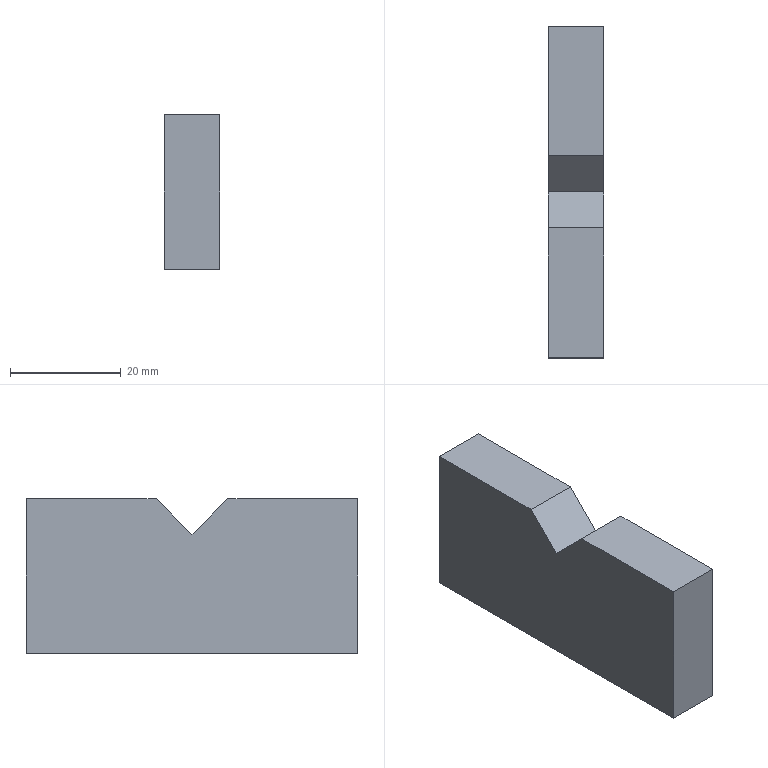Component | NX | REAR_BRACKET | 1 solid | 17 faces | box 10 x 60 x 28 mm | volume 15160 mm3 | plane 13 | cylinder 4 | commonest cylinder face diameters 5 x4
STEP:
#1=CARTESIAN_POINT('',(0.,0.,0.));
#2=DIRECTION('',(0.,0.,1.));
#3=DIRECTION('',(1.,0.,0.));
#4=AXIS2_PLACEMENT_3D('',#1,#2,#3);
#5=CARTESIAN_POINT('',(20.,-30.,34.5));
#6=VERTEX_POINT('',#5);
#7=CARTESIAN_POINT('',(20.,-6.5,34.5));
#8=VERTEX_POINT('',#7);
#9=CARTESIAN_POINT('',(20.,-30.,34.5));
#10=DIRECTION('',(0.,1.,-0.));
#11=VECTOR('',#10,1.);
#12=LINE('',#9,#11);
#13=CARTESIAN_POINT('',(30.,-30.,34.5));
#14=DIRECTION('',(0.,0.,1.));
#15=DIRECTION('',(0.,-1.,0.));
#16=AXIS2_PLACEMENT_3D('',#13,#14,#15);
#17=PLANE('',#16);
#18=CARTESIAN_POINT('',(0.,-10.));
#19=DIRECTION('',(-1.,0.));
#20=VECTOR('',#19,1.);
#21=LINE('',#18,#20);
#22=(GEOMETRIC_REPRESENTATION_CONTEXT(2)PARAMETRIC_REPRESENTATION_CONTEXT()REPRESENTATION_CONTEXT('',''));
#23=DEFINITIONAL_REPRESENTATION('',(#21),#22);
#24=PCURVE('',#17,#23);
#25=CARTESIAN_POINT('',(20.,0.,20.5));
#26=DIRECTION('',(-1.,0.,0.));
#27=DIRECTION('',(0.,0.,1.));
#28=AXIS2_PLACEMENT_3D('',#25,#26,#27);
#29=PLANE('',#28);
#30=CARTESIAN_POINT('',(14.,-30.));
#31=DIRECTION('',(-0.,1.));
#32=VECTOR('',#31,1.);
#33=LINE('',#30,#32);
#34=(GEOMETRIC_REPRESENTATION_CONTEXT(2)PARAMETRIC_REPRESENTATION_CONTEXT()REPRESENTATION_CONTEXT('',''));
#35=DEFINITIONAL_REPRESENTATION('',(#33),#34);
#36=PCURVE('',#29,#35);
#37=SURFACE_CURVE('',#12,(#24,#36),.PCURVE_S1.);
#38=EDGE_CURVE('',#6,#8,#37,.T.);
#39=ORIENTED_EDGE('',*,*,#38,.F.);
#40=CARTESIAN_POINT('',(30.,-30.,34.5));
#41=VERTEX_POINT('',#40);
#42=CARTESIAN_POINT('',(30.,-30.,34.5));
#43=DIRECTION('',(-1.,0.,0.));
#44=VECTOR('',#43,1.);
#45=LINE('',#42,#44);
#46=CARTESIAN_POINT('',(0.,0.));
#47=DIRECTION('',(0.,-1.));
#48=VECTOR('',#47,1.);
#49=LINE('',#46,#48);
#50=(GEOMETRIC_REPRESENTATION_CONTEXT(2)PARAMETRIC_REPRESENTATION_CONTEXT()REPRESENTATION_CONTEXT('',''));
#51=DEFINITIONAL_REPRESENTATION('',(#49),#50);
#52=PCURVE('',#17,#51);
#53=CARTESIAN_POINT('',(30.,-30.,6.5));
#54=DIRECTION('',(0.,-1.,0.));
#55=DIRECTION('',(0.,0.,-1.));
#56=AXIS2_PLACEMENT_3D('',#53,#54,#55);
#57=PLANE('',#56);
#58=CARTESIAN_POINT('',(-28.,0.));
#59=DIRECTION('',(0.,-1.));
#60=VECTOR('',#59,1.);
#61=LINE('',#58,#60);
#62=(GEOMETRIC_REPRESENTATION_CONTEXT(2)PARAMETRIC_REPRESENTATION_CONTEXT()REPRESENTATION_CONTEXT('',''));
#63=DEFINITIONAL_REPRESENTATION('',(#61),#62);
#64=PCURVE('',#57,#63);
#65=SURFACE_CURVE('',#45,(#52,#64),.PCURVE_S1.);
#66=EDGE_CURVE('',#41,#6,#65,.T.);
#67=ORIENTED_EDGE('',*,*,#66,.F.);
#68=CARTESIAN_POINT('',(30.,-6.5,34.5));
#69=VERTEX_POINT('',#68);
#70=CARTESIAN_POINT('',(30.,-30.,34.5));
#71=DIRECTION('',(0.,1.,-0.));
#72=VECTOR('',#71,1.);
#73=LINE('',#70,#72);
#74=CARTESIAN_POINT('',(0.,0.));
#75=DIRECTION('',(-1.,0.));
#76=VECTOR('',#75,1.);
#77=LINE('',#74,#76);
#78=(GEOMETRIC_REPRESENTATION_CONTEXT(2)PARAMETRIC_REPRESENTATION_CONTEXT()REPRESENTATION_CONTEXT('',''));
#79=DEFINITIONAL_REPRESENTATION('',(#77),#78);
#80=PCURVE('',#17,#79);
#81=CARTESIAN_POINT('',(30.,0.,20.5));
#82=DIRECTION('',(-1.,0.,0.));
#83=DIRECTION('',(0.,0.,1.));
#84=AXIS2_PLACEMENT_3D('',#81,#82,#83);
#85=PLANE('',#84);
#86=CARTESIAN_POINT('',(14.,-30.));
#87=DIRECTION('',(-0.,1.));
#88=VECTOR('',#87,1.);
#89=LINE('',#86,#88);
#90=(GEOMETRIC_REPRESENTATION_CONTEXT(2)PARAMETRIC_REPRESENTATION_CONTEXT()REPRESENTATION_CONTEXT('',''));
#91=DEFINITIONAL_REPRESENTATION('',(#89),#90);
#92=PCURVE('',#85,#91);
#93=SURFACE_CURVE('',#73,(#80,#92),.PCURVE_S1.);
#94=EDGE_CURVE('',#41,#69,#93,.T.);
#95=ORIENTED_EDGE('',*,*,#94,.T.);
#96=CARTESIAN_POINT('',(30.,-6.5,34.5));
#97=DIRECTION('',(-1.,0.,0.));
#98=VECTOR('',#97,1.);
#99=LINE('',#96,#98);
#100=CARTESIAN_POINT('',(-23.5,0.));
#101=DIRECTION('',(0.,-1.));
#102=VECTOR('',#101,1.);
#103=LINE('',#100,#102);
#104=(GEOMETRIC_REPRESENTATION_CONTEXT(2)PARAMETRIC_REPRESENTATION_CONTEXT()REPRESENTATION_CONTEXT('',''));
#105=DEFINITIONAL_REPRESENTATION('',(#103),#104);
#106=PCURVE('',#17,#105);
#107=CARTESIAN_POINT('',(30.,-6.5,34.5));
#108=DIRECTION('',(0.,0.7071,0.7071));
#109=DIRECTION('',(0.,-0.7071,0.7071));
#110=AXIS2_PLACEMENT_3D('',#107,#108,#109);
#111=PLANE('',#110);
#112=CARTESIAN_POINT('',(0.,0.));
#113=DIRECTION('',(0.,-1.));
#114=VECTOR('',#113,1.);
#115=LINE('',#112,#114);
#116=(GEOMETRIC_REPRESENTATION_CONTEXT(2)PARAMETRIC_REPRESENTATION_CONTEXT()REPRESENTATION_CONTEXT('',''));
#117=DEFINITIONAL_REPRESENTATION('',(#115),#116);
#118=PCURVE('',#111,#117);
#119=SURFACE_CURVE('',#99,(#106,#118),.PCURVE_S1.);
#120=EDGE_CURVE('',#69,#8,#119,.T.);
#121=ORIENTED_EDGE('',*,*,#120,.T.);
#122=EDGE_LOOP('',(#39,#67,#95,#121));
#123=FACE_BOUND('',#122,.T.);
#124=ADVANCED_FACE('',(#123),#17,.T.);
#125=CARTESIAN_POINT('',(20.,0.,28.));
#126=VERTEX_POINT('',#125);
#127=CARTESIAN_POINT('',(20.,-6.5,34.5));
#128=DIRECTION('',(0.,0.7071,-0.7071));
#129=VECTOR('',#128,1.);
#130=LINE('',#127,#129);
#131=CARTESIAN_POINT('',(0.,-10.));
#132=DIRECTION('',(-1.,0.));
#133=VECTOR('',#132,1.);
#134=LINE('',#131,#133);
#135=(GEOMETRIC_REPRESENTATION_CONTEXT(2)PARAMETRIC_REPRESENTATION_CONTEXT()REPRESENTATION_CONTEXT('',''));
#136=DEFINITIONAL_REPRESENTATION('',(#134),#135);
#137=PCURVE('',#111,#136);
#138=CARTESIAN_POINT('',(14.,-6.5));
#139=DIRECTION('',(-0.7071,0.7071));
#140=VECTOR('',#139,1.);
#141=LINE('',#138,#140);
#142=(GEOMETRIC_REPRESENTATION_CONTEXT(2)PARAMETRIC_REPRESENTATION_CONTEXT()REPRESENTATION_CONTEXT('',''));
#143=DEFINITIONAL_REPRESENTATION('',(#141),#142);
#144=PCURVE('',#29,#143);
#145=SURFACE_CURVE('',#130,(#137,#144),.PCURVE_S1.);
#146=EDGE_CURVE('',#8,#126,#145,.T.);
#147=ORIENTED_EDGE('',*,*,#146,.F.);
#148=ORIENTED_EDGE('',*,*,#120,.F.);
#149=CARTESIAN_POINT('',(30.,0.,28.));
#150=VERTEX_POINT('',#149);
#151=CARTESIAN_POINT('',(30.,-6.5,34.5));
#152=DIRECTION('',(0.,0.7071,-0.7071));
#153=VECTOR('',#152,1.);
#154=LINE('',#151,#153);
#155=CARTESIAN_POINT('',(0.,0.));
#156=DIRECTION('',(-1.,0.));
#157=VECTOR('',#156,1.);
#158=LINE('',#155,#157);
#159=(GEOMETRIC_REPRESENTATION_CONTEXT(2)PARAMETRIC_REPRESENTATION_CONTEXT()REPRESENTATION_CONTEXT('',''));
#160=DEFINITIONAL_REPRESENTATION('',(#158),#159);
#161=PCURVE('',#111,#160);
#162=CARTESIAN_POINT('',(14.,-6.5));
#163=DIRECTION('',(-0.7071,0.7071));
#164=VECTOR('',#163,1.);
#165=LINE('',#162,#164);
#166=(GEOMETRIC_REPRESENTATION_CONTEXT(2)PARAMETRIC_REPRESENTATION_CONTEXT()REPRESENTATION_CONTEXT('',''));
#167=DEFINITIONAL_REPRESENTATION('',(#165),#166);
#168=PCURVE('',#85,#167);
#169=SURFACE_CURVE('',#154,(#161,#168),.PCURVE_S1.);
#170=EDGE_CURVE('',#69,#150,#169,.T.);
#171=ORIENTED_EDGE('',*,*,#170,.T.);
#172=CARTESIAN_POINT('',(30.,0.,28.));
#173=DIRECTION('',(-1.,0.,0.));
#174=VECTOR('',#173,1.);
#175=LINE('',#172,#174);
#176=CARTESIAN_POINT('',(-9.192,0.));
#177=DIRECTION('',(0.,-1.));
#178=VECTOR('',#177,1.);
#179=LINE('',#176,#178);
#180=(GEOMETRIC_REPRESENTATION_CONTEXT(2)PARAMETRIC_REPRESENTATION_CONTEXT()REPRESENTATION_CONTEXT('',''));
#181=DEFINITIONAL_REPRESENTATION('',(#179),#180);
#182=PCURVE('',#111,#181);
#183=CARTESIAN_POINT('',(30.,0.,28.));
#184=DIRECTION('',(0.,-0.7071,0.7071));
#185=DIRECTION('',(0.,-0.7071,-0.7071));
#186=AXIS2_PLACEMENT_3D('',#183,#184,#185);
#187=PLANE('',#186);
#188=CARTESIAN_POINT('',(0.,0.));
#189=DIRECTION('',(0.,-1.));
#190=VECTOR('',#189,1.);
#191=LINE('',#188,#190);
#192=(GEOMETRIC_REPRESENTATION_CONTEXT(2)PARAMETRIC_REPRESENTATION_CONTEXT()REPRESENTATION_CONTEXT('',''));
#193=DEFINITIONAL_REPRESENTATION('',(#191),#192);
#194=PCURVE('',#187,#193);
#195=SURFACE_CURVE('',#175,(#182,#194),.PCURVE_S1.);
#196=EDGE_CURVE('',#150,#126,#195,.T.);
#197=ORIENTED_EDGE('',*,*,#196,.T.);
#198=EDGE_LOOP('',(#147,#148,#171,#197));
#199=FACE_BOUND('',#198,.T.);
#200=ADVANCED_FACE('',(#199),#111,.T.);
#201=CARTESIAN_POINT('',(20.,6.5,34.5));
#202=VERTEX_POINT('',#201);
#203=CARTESIAN_POINT('',(20.,0.,28.));
#204=DIRECTION('',(0.,0.7071,0.7071));
#205=VECTOR('',#204,1.);
#206=LINE('',#203,#205);
#207=CARTESIAN_POINT('',(0.,-10.));
#208=DIRECTION('',(-1.,0.));
#209=VECTOR('',#208,1.);
#210=LINE('',#207,#209);
#211=(GEOMETRIC_REPRESENTATION_CONTEXT(2)PARAMETRIC_REPRESENTATION_CONTEXT()REPRESENTATION_CONTEXT('',''));
#212=DEFINITIONAL_REPRESENTATION('',(#210),#211);
#213=PCURVE('',#187,#212);
#214=CARTESIAN_POINT('',(7.5,0.));
#215=DIRECTION('',(0.7071,0.7071));
#216=VECTOR('',#215,1.);
#217=LINE('',#214,#216);
#218=(GEOMETRIC_REPRESENTATION_CONTEXT(2)PARAMETRIC_REPRESENTATION_CONTEXT()REPRESENTATION_CONTEXT('',''));
#219=DEFINITIONAL_REPRESENTATION('',(#217),#218);
#220=PCURVE('',#29,#219);
#221=SURFACE_CURVE('',#206,(#213,#220),.PCURVE_S1.);
#222=EDGE_CURVE('',#126,#202,#221,.T.);
#223=ORIENTED_EDGE('',*,*,#222,.F.);
#224=ORIENTED_EDGE('',*,*,#196,.F.);
#225=CARTESIAN_POINT('',(30.,6.5,34.5));
#226=VERTEX_POINT('',#225);
#227=CARTESIAN_POINT('',(30.,0.,28.));
#228=DIRECTION('',(0.,0.7071,0.7071));
#229=VECTOR('',#228,1.);
#230=LINE('',#227,#229);
#231=CARTESIAN_POINT('',(0.,0.));
#232=DIRECTION('',(-1.,0.));
#233=VECTOR('',#232,1.);
#234=LINE('',#231,#233);
#235=(GEOMETRIC_REPRESENTATION_CONTEXT(2)PARAMETRIC_REPRESENTATION_CONTEXT()REPRESENTATION_CONTEXT('',''));
#236=DEFINITIONAL_REPRESENTATION('',(#234),#235);
#237=PCURVE('',#187,#236);
#238=CARTESIAN_POINT('',(7.5,0.));
#239=DIRECTION('',(0.7071,0.7071));
#240=VECTOR('',#239,1.);
#241=LINE('',#238,#240);
#242=(GEOMETRIC_REPRESENTATION_CONTEXT(2)PARAMETRIC_REPRESENTATION_CONTEXT()REPRESENTATION_CONTEXT('',''));
#243=DEFINITIONAL_REPRESENTATION('',(#241),#242);
#244=PCURVE('',#85,#243);
#245=SURFACE_CURVE('',#230,(#237,#244),.PCURVE_S1.);
#246=EDGE_CURVE('',#150,#226,#245,.T.);
#247=ORIENTED_EDGE('',*,*,#246,.T.);
#248=CARTESIAN_POINT('',(30.,6.5,34.5));
#249=DIRECTION('',(-1.,0.,0.));
#250=VECTOR('',#249,1.);
#251=LINE('',#248,#250);
#252=CARTESIAN_POINT('',(-9.192,0.));
#253=DIRECTION('',(0.,-1.));
#254=VECTOR('',#253,1.);
#255=LINE('',#252,#254);
#256=(GEOMETRIC_REPRESENTATION_CONTEXT(2)PARAMETRIC_REPRESENTATION_CONTEXT()REPRESENTATION_CONTEXT('',''));
#257=DEFINITIONAL_REPRESENTATION('',(#255),#256);
#258=PCURVE('',#187,#257);
#259=CARTESIAN_POINT('',(30.,6.5,34.5));
#260=DIRECTION('',(0.,-0.,1.));
#261=DIRECTION('',(0.,-1.,-0.));
#262=AXIS2_PLACEMENT_3D('',#259,#260,#261);
#263=PLANE('',#262);
#264=CARTESIAN_POINT('',(0.,0.));
#265=DIRECTION('',(0.,-1.));
#266=VECTOR('',#265,1.);
#267=LINE('',#264,#266);
#268=(GEOMETRIC_REPRESENTATION_CONTEXT(2)PARAMETRIC_REPRESENTATION_CONTEXT()REPRESENTATION_CONTEXT('',''));
#269=DEFINITIONAL_REPRESENTATION('',(#267),#268);
#270=PCURVE('',#263,#269);
#271=SURFACE_CURVE('',#251,(#258,#270),.PCURVE_S1.);
#272=EDGE_CURVE('',#226,#202,#271,.T.);
#273=ORIENTED_EDGE('',*,*,#272,.T.);
#274=EDGE_LOOP('',(#223,#224,#247,#273));
#275=FACE_BOUND('',#274,.T.);
#276=ADVANCED_FACE('',(#275),#187,.T.);
#277=CARTESIAN_POINT('',(20.,30.,34.5));
#278=VERTEX_POINT('',#277);
#279=CARTESIAN_POINT('',(20.,6.5,34.5));
#280=DIRECTION('',(0.,1.,0.));
#281=VECTOR('',#280,1.);
#282=LINE('',#279,#281);
#283=CARTESIAN_POINT('',(0.,-10.));
#284=DIRECTION('',(-1.,0.));
#285=VECTOR('',#284,1.);
#286=LINE('',#283,#285);
#287=(GEOMETRIC_REPRESENTATION_CONTEXT(2)PARAMETRIC_REPRESENTATION_CONTEXT()REPRESENTATION_CONTEXT('',''));
#288=DEFINITIONAL_REPRESENTATION('',(#286),#287);
#289=PCURVE('',#263,#288);
#290=CARTESIAN_POINT('',(14.,6.5));
#291=DIRECTION('',(0.,1.));
#292=VECTOR('',#291,1.);
#293=LINE('',#290,#292);
#294=(GEOMETRIC_REPRESENTATION_CONTEXT(2)PARAMETRIC_REPRESENTATION_CONTEXT()REPRESENTATION_CONTEXT('',''));
#295=DEFINITIONAL_REPRESENTATION('',(#293),#294);
#296=PCURVE('',#29,#295);
#297=SURFACE_CURVE('',#282,(#289,#296),.PCURVE_S1.);
#298=EDGE_CURVE('',#202,#278,#297,.T.);
#299=ORIENTED_EDGE('',*,*,#298,.F.);
#300=ORIENTED_EDGE('',*,*,#272,.F.);
#301=CARTESIAN_POINT('',(30.,30.,34.5));
#302=VERTEX_POINT('',#301);
#303=CARTESIAN_POINT('',(30.,6.5,34.5));
#304=DIRECTION('',(0.,1.,0.));
#305=VECTOR('',#304,1.);
#306=LINE('',#303,#305);
#307=CARTESIAN_POINT('',(0.,0.));
#308=DIRECTION('',(-1.,0.));
#309=VECTOR('',#308,1.);
#310=LINE('',#307,#309);
#311=(GEOMETRIC_REPRESENTATION_CONTEXT(2)PARAMETRIC_REPRESENTATION_CONTEXT()REPRESENTATION_CONTEXT('',''));
#312=DEFINITIONAL_REPRESENTATION('',(#310),#311);
#313=PCURVE('',#263,#312);
#314=CARTESIAN_POINT('',(14.,6.5));
#315=DIRECTION('',(0.,1.));
#316=VECTOR('',#315,1.);
#317=LINE('',#314,#316);
#318=(GEOMETRIC_REPRESENTATION_CONTEXT(2)PARAMETRIC_REPRESENTATION_CONTEXT()REPRESENTATION_CONTEXT('',''));
#319=DEFINITIONAL_REPRESENTATION('',(#317),#318);
#320=PCURVE('',#85,#319);
#321=SURFACE_CURVE('',#306,(#313,#320),.PCURVE_S1.);
#322=EDGE_CURVE('',#226,#302,#321,.T.);
#323=ORIENTED_EDGE('',*,*,#322,.T.);
#324=CARTESIAN_POINT('',(30.,30.,34.5));
#325=DIRECTION('',(-1.,0.,0.));
#326=VECTOR('',#325,1.);
#327=LINE('',#324,#326);
#328=CARTESIAN_POINT('',(-23.5,0.));
#329=DIRECTION('',(0.,-1.));
#330=VECTOR('',#329,1.);
#331=LINE('',#328,#330);
#332=(GEOMETRIC_REPRESENTATION_CONTEXT(2)PARAMETRIC_REPRESENTATION_CONTEXT()REPRESENTATION_CONTEXT('',''));
#333=DEFINITIONAL_REPRESENTATION('',(#331),#332);
#334=PCURVE('',#263,#333);
#335=CARTESIAN_POINT('',(30.,30.,34.5));
#336=DIRECTION('',(0.,1.,0.));
#337=DIRECTION('',(0.,0.,1.));
#338=AXIS2_PLACEMENT_3D('',#335,#336,#337);
#339=PLANE('',#338);
#340=CARTESIAN_POINT('',(0.,0.));
#341=DIRECTION('',(0.,-1.));
#342=VECTOR('',#341,1.);
#343=LINE('',#340,#342);
#344=(GEOMETRIC_REPRESENTATION_CONTEXT(2)PARAMETRIC_REPRESENTATION_CONTEXT()REPRESENTATION_CONTEXT('',''));
#345=DEFINITIONAL_REPRESENTATION('',(#343),#344);
#346=PCURVE('',#339,#345);
#347=SURFACE_CURVE('',#327,(#334,#346),.PCURVE_S1.);
#348=EDGE_CURVE('',#302,#278,#347,.T.);
#349=ORIENTED_EDGE('',*,*,#348,.T.);
#350=EDGE_LOOP('',(#299,#300,#323,#349));
#351=FACE_BOUND('',#350,.T.);
#352=ADVANCED_FACE('',(#351),#263,.T.);
#353=CARTESIAN_POINT('',(20.,30.,6.5));
#354=VERTEX_POINT('',#353);
#355=CARTESIAN_POINT('',(20.,30.,34.5));
#356=DIRECTION('',(0.,0.,-1.));
#357=VECTOR('',#356,1.);
#358=LINE('',#355,#357);
#359=CARTESIAN_POINT('',(0.,-10.));
#360=DIRECTION('',(-1.,0.));
#361=VECTOR('',#360,1.);
#362=LINE('',#359,#361);
#363=(GEOMETRIC_REPRESENTATION_CONTEXT(2)PARAMETRIC_REPRESENTATION_CONTEXT()REPRESENTATION_CONTEXT('',''));
#364=DEFINITIONAL_REPRESENTATION('',(#362),#363);
#365=PCURVE('',#339,#364);
#366=CARTESIAN_POINT('',(14.,30.));
#367=DIRECTION('',(-1.,0.));
#368=VECTOR('',#367,1.);
#369=LINE('',#366,#368);
#370=(GEOMETRIC_REPRESENTATION_CONTEXT(2)PARAMETRIC_REPRESENTATION_CONTEXT()REPRESENTATION_CONTEXT('',''));
#371=DEFINITIONAL_REPRESENTATION('',(#369),#370);
#372=PCURVE('',#29,#371);
#373=SURFACE_CURVE('',#358,(#365,#372),.PCURVE_S1.);
#374=EDGE_CURVE('',#278,#354,#373,.T.);
#375=ORIENTED_EDGE('',*,*,#374,.F.);
#376=ORIENTED_EDGE('',*,*,#348,.F.);
#377=CARTESIAN_POINT('',(30.,30.,6.5));
#378=VERTEX_POINT('',#377);
#379=CARTESIAN_POINT('',(30.,30.,34.5));
#380=DIRECTION('',(0.,0.,-1.));
#381=VECTOR('',#380,1.);
#382=LINE('',#379,#381);
#383=CARTESIAN_POINT('',(0.,0.));
#384=DIRECTION('',(-1.,0.));
#385=VECTOR('',#384,1.);
#386=LINE('',#383,#385);
#387=(GEOMETRIC_REPRESENTATION_CONTEXT(2)PARAMETRIC_REPRESENTATION_CONTEXT()REPRESENTATION_CONTEXT('',''));
#388=DEFINITIONAL_REPRESENTATION('',(#386),#387);
#389=PCURVE('',#339,#388);
#390=CARTESIAN_POINT('',(14.,30.));
#391=DIRECTION('',(-1.,0.));
#392=VECTOR('',#391,1.);
#393=LINE('',#390,#392);
#394=(GEOMETRIC_REPRESENTATION_CONTEXT(2)PARAMETRIC_REPRESENTATION_CONTEXT()REPRESENTATION_CONTEXT('',''));
#395=DEFINITIONAL_REPRESENTATION('',(#393),#394);
#396=PCURVE('',#85,#395);
#397=SURFACE_CURVE('',#382,(#389,#396),.PCURVE_S1.);
#398=EDGE_CURVE('',#302,#378,#397,.T.);
#399=ORIENTED_EDGE('',*,*,#398,.T.);
#400=CARTESIAN_POINT('',(30.,30.,6.5));
#401=DIRECTION('',(-1.,0.,0.));
#402=VECTOR('',#401,1.);
#403=LINE('',#400,#402);
#404=CARTESIAN_POINT('',(-28.,0.));
#405=DIRECTION('',(0.,-1.));
#406=VECTOR('',#405,1.);
#407=LINE('',#404,#406);
#408=(GEOMETRIC_REPRESENTATION_CONTEXT(2)PARAMETRIC_REPRESENTATION_CONTEXT()REPRESENTATION_CONTEXT('',''));
#409=DEFINITIONAL_REPRESENTATION('',(#407),#408);
#410=PCURVE('',#339,#409);
#411=CARTESIAN_POINT('',(30.,30.,6.5));
#412=DIRECTION('',(0.,0.,-1.));
#413=DIRECTION('',(-1.,0.,0.));
#414=AXIS2_PLACEMENT_3D('',#411,#412,#413);
#415=PLANE('',#414);
#416=CARTESIAN_POINT('',(0.,0.));
#417=DIRECTION('',(1.,0.));
#418=VECTOR('',#417,1.);
#419=LINE('',#416,#418);
#420=(GEOMETRIC_REPRESENTATION_CONTEXT(2)PARAMETRIC_REPRESENTATION_CONTEXT()REPRESENTATION_CONTEXT('',''));
#421=DEFINITIONAL_REPRESENTATION('',(#419),#420);
#422=PCURVE('',#415,#421);
#423=SURFACE_CURVE('',#403,(#410,#422),.PCURVE_S1.);
#424=EDGE_CURVE('',#378,#354,#423,.T.);
#425=ORIENTED_EDGE('',*,*,#424,.T.);
#426=EDGE_LOOP('',(#375,#376,#399,#425));
#427=FACE_BOUND('',#426,.T.);
#428=ADVANCED_FACE('',(#427),#339,.T.);
#429=CARTESIAN_POINT('',(25.,-17.5,6.5));
#430=VERTEX_POINT('',#429);
#431=CARTESIAN_POINT('',(25.,-20.,6.5));
#432=DIRECTION('',(0.,0.,-1.));
#433=DIRECTION('',(0.,1.,0.));
#434=AXIS2_PLACEMENT_3D('',#431,#432,#433);
#435=CIRCLE('',#434,2.5);
#436=CARTESIAN_POINT('',(5.,-50.));
#437=DIRECTION('',(0.,1.));
#438=AXIS2_PLACEMENT_2D('',#436,#437);
#439=CIRCLE('',#438,2.5);
#440=(GEOMETRIC_REPRESENTATION_CONTEXT(2)PARAMETRIC_REPRESENTATION_CONTEXT()REPRESENTATION_CONTEXT('',''));
#441=DEFINITIONAL_REPRESENTATION('',(#439),#440);
#442=PCURVE('',#415,#441);
#443=CARTESIAN_POINT('',(25.,-20.,24.5));
#444=DIRECTION('',(0.,0.,-1.));
#445=DIRECTION('',(-1.,0.,0.));
#446=AXIS2_PLACEMENT_3D('',#443,#444,#445);
#447=CYLINDRICAL_SURFACE('',#446,2.5);
#448=CARTESIAN_POINT('',(1.571,18.));
#449=DIRECTION('',(1.,0.));
#450=VECTOR('',#449,1.);
#451=LINE('',#448,#450);
#452=(GEOMETRIC_REPRESENTATION_CONTEXT(2)PARAMETRIC_REPRESENTATION_CONTEXT()REPRESENTATION_CONTEXT('',''));
#453=DEFINITIONAL_REPRESENTATION('',(#451),#452);
#454=PCURVE('',#447,#453);
#455=SURFACE_CURVE('',#435,(#442,#454),.PCURVE_S1.);
#456=EDGE_CURVE('',#430,#430,#455,.T.);
#457=ORIENTED_EDGE('',*,*,#456,.F.);
#458=EDGE_LOOP('',(#457));
#459=FACE_BOUND('',#458,.T.);
#460=CARTESIAN_POINT('',(25.,17.5,6.5));
#461=VERTEX_POINT('',#460);
#462=CARTESIAN_POINT('',(25.,20.,6.5));
#463=DIRECTION('',(0.,0.,-1.));
#464=DIRECTION('',(0.,-1.,0.));
#465=AXIS2_PLACEMENT_3D('',#462,#463,#464);
#466=CIRCLE('',#465,2.5);
#467=CARTESIAN_POINT('',(5.,-10.));
#468=DIRECTION('',(0.,-1.));
#469=AXIS2_PLACEMENT_2D('',#467,#468);
#470=CIRCLE('',#469,2.5);
#471=(GEOMETRIC_REPRESENTATION_CONTEXT(2)PARAMETRIC_REPRESENTATION_CONTEXT()REPRESENTATION_CONTEXT('',''));
#472=DEFINITIONAL_REPRESENTATION('',(#470),#471);
#473=PCURVE('',#415,#472);
#474=CARTESIAN_POINT('',(25.,20.,24.5));
#475=DIRECTION('',(0.,0.,-1.));
#476=DIRECTION('',(-1.,0.,0.));
#477=AXIS2_PLACEMENT_3D('',#474,#475,#476);
#478=CYLINDRICAL_SURFACE('',#477,2.5);
#479=CARTESIAN_POINT('',(4.712,18.));
#480=DIRECTION('',(1.,0.));
#481=VECTOR('',#480,1.);
#482=LINE('',#479,#481);
#483=(GEOMETRIC_REPRESENTATION_CONTEXT(2)PARAMETRIC_REPRESENTATION_CONTEXT()REPRESENTATION_CONTEXT('',''));
#484=DEFINITIONAL_REPRESENTATION('',(#482),#483);
#485=PCURVE('',#478,#484);
#486=SURFACE_CURVE('',#466,(#473,#485),.PCURVE_S1.);
#487=EDGE_CURVE('',#461,#461,#486,.T.);
#488=ORIENTED_EDGE('',*,*,#487,.F.);
#489=EDGE_LOOP('',(#488));
#490=FACE_BOUND('',#489,.T.);
#491=CARTESIAN_POINT('',(25.,-8.5,6.5));
#492=VERTEX_POINT('',#491);
#493=CARTESIAN_POINT('',(25.,-11.,6.5));
#494=DIRECTION('',(0.,0.,-1.));
#495=DIRECTION('',(0.,1.,0.));
#496=AXIS2_PLACEMENT_3D('',#493,#494,#495);
#497=CIRCLE('',#496,2.5);
#498=CARTESIAN_POINT('',(5.,-41.));
#499=DIRECTION('',(0.,1.));
#500=AXIS2_PLACEMENT_2D('',#498,#499);
#501=CIRCLE('',#500,2.5);
#502=(GEOMETRIC_REPRESENTATION_CONTEXT(2)PARAMETRIC_REPRESENTATION_CONTEXT()REPRESENTATION_CONTEXT('',''));
#503=DEFINITIONAL_REPRESENTATION('',(#501),#502);
#504=PCURVE('',#415,#503);
#505=CARTESIAN_POINT('',(25.,-11.,19.5));
#506=DIRECTION('',(0.,0.,-1.));
#507=DIRECTION('',(-1.,0.,0.));
#508=AXIS2_PLACEMENT_3D('',#505,#506,#507);
#509=CYLINDRICAL_SURFACE('',#508,2.5);
#510=CARTESIAN_POINT('',(1.571,13.));
#511=DIRECTION('',(1.,0.));
#512=VECTOR('',#511,1.);
#513=LINE('',#510,#512);
#514=(GEOMETRIC_REPRESENTATION_CONTEXT(2)PARAMETRIC_REPRESENTATION_CONTEXT()REPRESENTATION_CONTEXT('',''));
#515=DEFINITIONAL_REPRESENTATION('',(#513),#514);
#516=PCURVE('',#509,#515);
#517=SURFACE_CURVE('',#497,(#504,#516),.PCURVE_S1.);
#518=EDGE_CURVE('',#492,#492,#517,.T.);
#519=ORIENTED_EDGE('',*,*,#518,.F.);
#520=EDGE_LOOP('',(#519));
#521=FACE_BOUND('',#520,.T.);
#522=CARTESIAN_POINT('',(25.,8.5,6.5));
#523=VERTEX_POINT('',#522);
#524=CARTESIAN_POINT('',(25.,11.,6.5));
#525=DIRECTION('',(0.,0.,-1.));
#526=DIRECTION('',(0.,-1.,0.));
#527=AXIS2_PLACEMENT_3D('',#524,#525,#526);
#528=CIRCLE('',#527,2.5);
#529=CARTESIAN_POINT('',(5.,-19.));
#530=DIRECTION('',(0.,-1.));
#531=AXIS2_PLACEMENT_2D('',#529,#530);
#532=CIRCLE('',#531,2.5);
#533=(GEOMETRIC_REPRESENTATION_CONTEXT(2)PARAMETRIC_REPRESENTATION_CONTEXT()REPRESENTATION_CONTEXT('',''));
#534=DEFINITIONAL_REPRESENTATION('',(#532),#533);
#535=PCURVE('',#415,#534);
#536=CARTESIAN_POINT('',(25.,11.,19.5));
#537=DIRECTION('',(0.,0.,-1.));
#538=DIRECTION('',(-1.,0.,0.));
#539=AXIS2_PLACEMENT_3D('',#536,#537,#538);
#540=CYLINDRICAL_SURFACE('',#539,2.5);
#541=CARTESIAN_POINT('',(4.712,13.));
#542=DIRECTION('',(1.,0.));
#543=VECTOR('',#542,1.);
#544=LINE('',#541,#543);
#545=(GEOMETRIC_REPRESENTATION_CONTEXT(2)PARAMETRIC_REPRESENTATION_CONTEXT()REPRESENTATION_CONTEXT('',''));
#546=DEFINITIONAL_REPRESENTATION('',(#544),#545);
#547=PCURVE('',#540,#546);
#548=SURFACE_CURVE('',#528,(#535,#547),.PCURVE_S1.);
#549=EDGE_CURVE('',#523,#523,#548,.T.);
#550=ORIENTED_EDGE('',*,*,#549,.F.);
#551=EDGE_LOOP('',(#550));
#552=FACE_BOUND('',#551,.T.);
#553=CARTESIAN_POINT('',(20.,-30.,6.5));
#554=VERTEX_POINT('',#553);
#555=CARTESIAN_POINT('',(20.,30.,6.5));
#556=DIRECTION('',(0.,-1.,0.));
#557=VECTOR('',#556,1.);
#558=LINE('',#555,#557);
#559=CARTESIAN_POINT('',(10.,0.));
#560=DIRECTION('',(0.,-1.));
#561=VECTOR('',#560,1.);
#562=LINE('',#559,#561);
#563=(GEOMETRIC_REPRESENTATION_CONTEXT(2)PARAMETRIC_REPRESENTATION_CONTEXT()REPRESENTATION_CONTEXT('',''));
#564=DEFINITIONAL_REPRESENTATION('',(#562),#563);
#565=PCURVE('',#415,#564);
#566=CARTESIAN_POINT('',(-14.,30.));
#567=DIRECTION('',(0.,-1.));
#568=VECTOR('',#567,1.);
#569=LINE('',#566,#568);
#570=(GEOMETRIC_REPRESENTATION_CONTEXT(2)PARAMETRIC_REPRESENTATION_CONTEXT()REPRESENTATION_CONTEXT('',''));
#571=DEFINITIONAL_REPRESENTATION('',(#569),#570);
#572=PCURVE('',#29,#571);
#573=SURFACE_CURVE('',#558,(#565,#572),.PCURVE_S1.);
#574=EDGE_CURVE('',#354,#554,#573,.T.);
#575=ORIENTED_EDGE('',*,*,#574,.F.);
#576=ORIENTED_EDGE('',*,*,#424,.F.);
#577=CARTESIAN_POINT('',(30.,-30.,6.5));
#578=VERTEX_POINT('',#577);
#579=CARTESIAN_POINT('',(30.,30.,6.5));
#580=DIRECTION('',(0.,-1.,0.));
#581=VECTOR('',#580,1.);
#582=LINE('',#579,#581);
#583=CARTESIAN_POINT('',(0.,0.));
#584=DIRECTION('',(0.,-1.));
#585=VECTOR('',#584,1.);
#586=LINE('',#583,#585);
#587=(GEOMETRIC_REPRESENTATION_CONTEXT(2)PARAMETRIC_REPRESENTATION_CONTEXT()REPRESENTATION_CONTEXT('',''));
#588=DEFINITIONAL_REPRESENTATION('',(#586),#587);
#589=PCURVE('',#415,#588);
#590=CARTESIAN_POINT('',(-14.,30.));
#591=DIRECTION('',(0.,-1.));
#592=VECTOR('',#591,1.);
#593=LINE('',#590,#592);
#594=(GEOMETRIC_REPRESENTATION_CONTEXT(2)PARAMETRIC_REPRESENTATION_CONTEXT()REPRESENTATION_CONTEXT('',''));
#595=DEFINITIONAL_REPRESENTATION('',(#593),#594);
#596=PCURVE('',#85,#595);
#597=SURFACE_CURVE('',#582,(#589,#596),.PCURVE_S1.);
#598=EDGE_CURVE('',#378,#578,#597,.T.);
#599=ORIENTED_EDGE('',*,*,#598,.T.);
#600=CARTESIAN_POINT('',(30.,-30.,6.5));
#601=DIRECTION('',(-1.,0.,0.));
#602=VECTOR('',#601,1.);
#603=LINE('',#600,#602);
#604=CARTESIAN_POINT('',(0.,-60.));
#605=DIRECTION('',(1.,0.));
#606=VECTOR('',#605,1.);
#607=LINE('',#604,#606);
#608=(GEOMETRIC_REPRESENTATION_CONTEXT(2)PARAMETRIC_REPRESENTATION_CONTEXT()REPRESENTATION_CONTEXT('',''));
#609=DEFINITIONAL_REPRESENTATION('',(#607),#608);
#610=PCURVE('',#415,#609);
#611=CARTESIAN_POINT('',(0.,0.));
#612=DIRECTION('',(0.,-1.));
#613=VECTOR('',#612,1.);
#614=LINE('',#611,#613);
#615=(GEOMETRIC_REPRESENTATION_CONTEXT(2)PARAMETRIC_REPRESENTATION_CONTEXT()REPRESENTATION_CONTEXT('',''));
#616=DEFINITIONAL_REPRESENTATION('',(#614),#615);
#617=PCURVE('',#57,#616);
#618=SURFACE_CURVE('',#603,(#610,#617),.PCURVE_S1.);
#619=EDGE_CURVE('',#578,#554,#618,.T.);
#620=ORIENTED_EDGE('',*,*,#619,.T.);
#621=EDGE_LOOP('',(#575,#576,#599,#620));
#622=FACE_BOUND('',#621,.T.);
#623=ADVANCED_FACE('',(#459,#490,#521,#552,#622),#415,.T.);
#624=CARTESIAN_POINT('',(20.,-30.,6.5));
#625=DIRECTION('',(0.,0.,1.));
#626=VECTOR('',#625,1.);
#627=LINE('',#624,#626);
#628=CARTESIAN_POINT('',(0.,-10.));
#629=DIRECTION('',(-1.,0.));
#630=VECTOR('',#629,1.);
#631=LINE('',#628,#630);
#632=(GEOMETRIC_REPRESENTATION_CONTEXT(2)PARAMETRIC_REPRESENTATION_CONTEXT()REPRESENTATION_CONTEXT('',''));
#633=DEFINITIONAL_REPRESENTATION('',(#631),#632);
#634=PCURVE('',#57,#633);
#635=CARTESIAN_POINT('',(-14.,-30.));
#636=DIRECTION('',(1.,0.));
#637=VECTOR('',#636,1.);
#638=LINE('',#635,#637);
#639=(GEOMETRIC_REPRESENTATION_CONTEXT(2)PARAMETRIC_REPRESENTATION_CONTEXT()REPRESENTATION_CONTEXT('',''));
#640=DEFINITIONAL_REPRESENTATION('',(#638),#639);
#641=PCURVE('',#29,#640);
#642=SURFACE_CURVE('',#627,(#634,#641),.PCURVE_S1.);
#643=EDGE_CURVE('',#554,#6,#642,.T.);
#644=ORIENTED_EDGE('',*,*,#643,.F.);
#645=ORIENTED_EDGE('',*,*,#619,.F.);
#646=CARTESIAN_POINT('',(30.,-30.,6.5));
#647=DIRECTION('',(0.,0.,1.));
#648=VECTOR('',#647,1.);
#649=LINE('',#646,#648);
#650=CARTESIAN_POINT('',(0.,0.));
#651=DIRECTION('',(-1.,0.));
#652=VECTOR('',#651,1.);
#653=LINE('',#650,#652);
#654=(GEOMETRIC_REPRESENTATION_CONTEXT(2)PARAMETRIC_REPRESENTATION_CONTEXT()REPRESENTATION_CONTEXT('',''));
#655=DEFINITIONAL_REPRESENTATION('',(#653),#654);
#656=PCURVE('',#57,#655);
#657=CARTESIAN_POINT('',(-14.,-30.));
#658=DIRECTION('',(1.,0.));
#659=VECTOR('',#658,1.);
#660=LINE('',#657,#659);
#661=(GEOMETRIC_REPRESENTATION_CONTEXT(2)PARAMETRIC_REPRESENTATION_CONTEXT()REPRESENTATION_CONTEXT('',''));
#662=DEFINITIONAL_REPRESENTATION('',(#660),#661);
#663=PCURVE('',#85,#662);
#664=SURFACE_CURVE('',#649,(#656,#663),.PCURVE_S1.);
#665=EDGE_CURVE('',#578,#41,#664,.T.);
#666=ORIENTED_EDGE('',*,*,#665,.T.);
#667=ORIENTED_EDGE('',*,*,#66,.T.);
#668=EDGE_LOOP('',(#644,#645,#666,#667));
#669=FACE_BOUND('',#668,.T.);
#670=ADVANCED_FACE('',(#669),#57,.T.);
#671=ORIENTED_EDGE('',*,*,#94,.F.);
#672=ORIENTED_EDGE('',*,*,#665,.F.);
#673=ORIENTED_EDGE('',*,*,#598,.F.);
#674=ORIENTED_EDGE('',*,*,#398,.F.);
#675=ORIENTED_EDGE('',*,*,#322,.F.);
#676=ORIENTED_EDGE('',*,*,#246,.F.);
#677=ORIENTED_EDGE('',*,*,#170,.F.);
#678=EDGE_LOOP('',(#671,#672,#673,#674,#675,#676,#677));
#679=FACE_BOUND('',#678,.T.);
#680=ADVANCED_FACE('',(#679),#85,.F.);
#681=ORIENTED_EDGE('',*,*,#38,.T.);
#682=ORIENTED_EDGE('',*,*,#146,.T.);
#683=ORIENTED_EDGE('',*,*,#222,.T.);
#684=ORIENTED_EDGE('',*,*,#298,.T.);
#685=ORIENTED_EDGE('',*,*,#374,.T.);
#686=ORIENTED_EDGE('',*,*,#574,.T.);
#687=ORIENTED_EDGE('',*,*,#643,.T.);
#688=EDGE_LOOP('',(#681,#682,#683,#684,#685,#686,#687));
#689=FACE_BOUND('',#688,.T.);
#690=ADVANCED_FACE('',(#689),#29,.T.);
#691=CARTESIAN_POINT('',(25.,8.5,19.5));
#692=VERTEX_POINT('',#691);
#693=CARTESIAN_POINT('',(25.,11.,19.5));
#694=DIRECTION('',(0.,0.,1.));
#695=DIRECTION('',(0.,-1.,0.));
#696=AXIS2_PLACEMENT_3D('',#693,#694,#695);
#697=CIRCLE('',#696,2.5);
#698=CARTESIAN_POINT('',(10.996,0.));
#699=DIRECTION('',(-1.,0.));
#700=VECTOR('',#699,1.);
#701=LINE('',#698,#700);
#702=(GEOMETRIC_REPRESENTATION_CONTEXT(2)PARAMETRIC_REPRESENTATION_CONTEXT()REPRESENTATION_CONTEXT('',''));
#703=DEFINITIONAL_REPRESENTATION('',(#701),#702);
#704=PCURVE('',#540,#703);
#705=CARTESIAN_POINT('',(25.,11.,19.5));
#706=DIRECTION('',(0.,0.,-1.));
#707=DIRECTION('',(-1.,0.,0.));
#708=AXIS2_PLACEMENT_3D('',#705,#706,#707);
#709=PLANE('',#708);
#710=CARTESIAN_POINT('',(0.,-2.5));
#711=CARTESIAN_POINT('',(-4.33,-2.5));
#712=CARTESIAN_POINT('',(-2.165,1.25));
#713=CARTESIAN_POINT('',(-0.,5.));
#714=CARTESIAN_POINT('',(2.165,1.25));
#715=CARTESIAN_POINT('',(4.33,-2.5));
#716=CARTESIAN_POINT('',(0.,-2.5));
#717=(BOUNDED_CURVE()B_SPLINE_CURVE(2,(#710,#711,#712,#713,#714,#715,#716),.UNSPECIFIED.,.T.,.F.)B_SPLINE_CURVE_WITH_KNOTS((1,2,2,2,2,1),(-2.094,0.,2.094,4.189,6.283,8.378),.UNSPECIFIED.)CURVE()GEOMETRIC_REPRESENTATION_ITEM()RATIONAL_B_SPLINE_CURVE((1.,0.5,1.,0.5,1.,0.5,1.))REPRESENTATION_ITEM(''));
#718=(GEOMETRIC_REPRESENTATION_CONTEXT(2)PARAMETRIC_REPRESENTATION_CONTEXT()REPRESENTATION_CONTEXT('',''));
#719=DEFINITIONAL_REPRESENTATION('',(#717),#718);
#720=PCURVE('',#709,#719);
#721=SURFACE_CURVE('',#697,(#704,#720),.PCURVE_S1.);
#722=EDGE_CURVE('',#692,#692,#721,.T.);
#723=ORIENTED_EDGE('',*,*,#722,.F.);
#724=CARTESIAN_POINT('',(25.,8.5,19.5));
#725=CARTESIAN_POINT('',(25.,8.5,6.5));
#726=B_SPLINE_CURVE_WITH_KNOTS('',1,(#724,#725),.UNSPECIFIED.,.F.,.F.,(2,2),(0.,13.),.PIECEWISE_BEZIER_KNOTS.);
#727=CARTESIAN_POINT('',(10.996,0.));
#728=DIRECTION('',(0.,1.));
#729=VECTOR('',#728,1.);
#730=LINE('',#727,#729);
#731=(GEOMETRIC_REPRESENTATION_CONTEXT(2)PARAMETRIC_REPRESENTATION_CONTEXT()REPRESENTATION_CONTEXT('',''));
#732=DEFINITIONAL_REPRESENTATION('',(#730),#731);
#733=PCURVE('',#540,#732);
#734=CARTESIAN_POINT('',(4.712,0.));
#735=DIRECTION('',(0.,1.));
#736=VECTOR('',#735,1.);
#737=LINE('',#734,#736);
#738=(GEOMETRIC_REPRESENTATION_CONTEXT(2)PARAMETRIC_REPRESENTATION_CONTEXT()REPRESENTATION_CONTEXT('',''));
#739=DEFINITIONAL_REPRESENTATION('',(#737),#738);
#740=PCURVE('',#540,#739);
#741=SEAM_CURVE('',#726,(#733,#740),.PCURVE_S1.);
#742=EDGE_CURVE('',#692,#523,#741,.T.);
#743=ORIENTED_EDGE('',*,*,#742,.T.);
#744=ORIENTED_EDGE('',*,*,#549,.F.);
#745=ORIENTED_EDGE('',*,*,#742,.F.);
#746=EDGE_LOOP('',(#723,#743,#744,#745));
#747=FACE_BOUND('',#746,.F.);
#748=ADVANCED_FACE('',(#747),#540,.F.);
#749=ORIENTED_EDGE('',*,*,#722,.F.);
#750=EDGE_LOOP('',(#749));
#751=FACE_BOUND('',#750,.T.);
#752=ADVANCED_FACE('',(#751),#709,.T.);
#753=CARTESIAN_POINT('',(25.,-8.5,19.5));
#754=VERTEX_POINT('',#753);
#755=CARTESIAN_POINT('',(25.,-11.,19.5));
#756=DIRECTION('',(0.,0.,1.));
#757=DIRECTION('',(0.,1.,0.));
#758=AXIS2_PLACEMENT_3D('',#755,#756,#757);
#759=CIRCLE('',#758,2.5);
#760=CARTESIAN_POINT('',(7.854,0.));
#761=DIRECTION('',(-1.,0.));
#762=VECTOR('',#761,1.);
#763=LINE('',#760,#762);
#764=(GEOMETRIC_REPRESENTATION_CONTEXT(2)PARAMETRIC_REPRESENTATION_CONTEXT()REPRESENTATION_CONTEXT('',''));
#765=DEFINITIONAL_REPRESENTATION('',(#763),#764);
#766=PCURVE('',#509,#765);
#767=CARTESIAN_POINT('',(25.,-11.,19.5));
#768=DIRECTION('',(0.,0.,-1.));
#769=DIRECTION('',(-1.,0.,0.));
#770=AXIS2_PLACEMENT_3D('',#767,#768,#769);
#771=PLANE('',#770);
#772=CARTESIAN_POINT('',(0.,2.5));
#773=CARTESIAN_POINT('',(4.33,2.5));
#774=CARTESIAN_POINT('',(2.165,-1.25));
#775=CARTESIAN_POINT('',(0.,-5.));
#776=CARTESIAN_POINT('',(-2.165,-1.25));
#777=CARTESIAN_POINT('',(-4.33,2.5));
#778=CARTESIAN_POINT('',(0.,2.5));
#779=(BOUNDED_CURVE()B_SPLINE_CURVE(2,(#772,#773,#774,#775,#776,#777,#778),.UNSPECIFIED.,.T.,.F.)B_SPLINE_CURVE_WITH_KNOTS((1,2,2,2,2,1),(-2.094,0.,2.094,4.189,6.283,8.378),.UNSPECIFIED.)CURVE()GEOMETRIC_REPRESENTATION_ITEM()RATIONAL_B_SPLINE_CURVE((1.,0.5,1.,0.5,1.,0.5,1.))REPRESENTATION_ITEM(''));
#780=(GEOMETRIC_REPRESENTATION_CONTEXT(2)PARAMETRIC_REPRESENTATION_CONTEXT()REPRESENTATION_CONTEXT('',''));
#781=DEFINITIONAL_REPRESENTATION('',(#779),#780);
#782=PCURVE('',#771,#781);
#783=SURFACE_CURVE('',#759,(#766,#782),.PCURVE_S1.);
#784=EDGE_CURVE('',#754,#754,#783,.T.);
#785=ORIENTED_EDGE('',*,*,#784,.F.);
#786=CARTESIAN_POINT('',(25.,-8.5,19.5));
#787=CARTESIAN_POINT('',(25.,-8.5,6.5));
#788=B_SPLINE_CURVE_WITH_KNOTS('',1,(#786,#787),.UNSPECIFIED.,.F.,.F.,(2,2),(0.,13.),.PIECEWISE_BEZIER_KNOTS.);
#789=CARTESIAN_POINT('',(7.854,0.));
#790=DIRECTION('',(0.,1.));
#791=VECTOR('',#790,1.);
#792=LINE('',#789,#791);
#793=(GEOMETRIC_REPRESENTATION_CONTEXT(2)PARAMETRIC_REPRESENTATION_CONTEXT()REPRESENTATION_CONTEXT('',''));
#794=DEFINITIONAL_REPRESENTATION('',(#792),#793);
#795=PCURVE('',#509,#794);
#796=CARTESIAN_POINT('',(1.571,0.));
#797=DIRECTION('',(0.,1.));
#798=VECTOR('',#797,1.);
#799=LINE('',#796,#798);
#800=(GEOMETRIC_REPRESENTATION_CONTEXT(2)PARAMETRIC_REPRESENTATION_CONTEXT()REPRESENTATION_CONTEXT('',''));
#801=DEFINITIONAL_REPRESENTATION('',(#799),#800);
#802=PCURVE('',#509,#801);
#803=SEAM_CURVE('',#788,(#795,#802),.PCURVE_S1.);
#804=EDGE_CURVE('',#754,#492,#803,.T.);
#805=ORIENTED_EDGE('',*,*,#804,.T.);
#806=ORIENTED_EDGE('',*,*,#518,.F.);
#807=ORIENTED_EDGE('',*,*,#804,.F.);
#808=EDGE_LOOP('',(#785,#805,#806,#807));
#809=FACE_BOUND('',#808,.F.);
#810=ADVANCED_FACE('',(#809),#509,.F.);
#811=ORIENTED_EDGE('',*,*,#784,.F.);
#812=EDGE_LOOP('',(#811));
#813=FACE_BOUND('',#812,.T.);
#814=ADVANCED_FACE('',(#813),#771,.T.);
#815=CARTESIAN_POINT('',(25.,17.5,24.5));
#816=VERTEX_POINT('',#815);
#817=CARTESIAN_POINT('',(25.,20.,24.5));
#818=DIRECTION('',(0.,0.,1.));
#819=DIRECTION('',(0.,-1.,0.));
#820=AXIS2_PLACEMENT_3D('',#817,#818,#819);
#821=CIRCLE('',#820,2.5);
#822=CARTESIAN_POINT('',(10.996,0.));
#823=DIRECTION('',(-1.,0.));
#824=VECTOR('',#823,1.);
#825=LINE('',#822,#824);
#826=(GEOMETRIC_REPRESENTATION_CONTEXT(2)PARAMETRIC_REPRESENTATION_CONTEXT()REPRESENTATION_CONTEXT('',''));
#827=DEFINITIONAL_REPRESENTATION('',(#825),#826);
#828=PCURVE('',#478,#827);
#829=CARTESIAN_POINT('',(25.,20.,24.5));
#830=DIRECTION('',(0.,0.,-1.));
#831=DIRECTION('',(-1.,0.,0.));
#832=AXIS2_PLACEMENT_3D('',#829,#830,#831);
#833=PLANE('',#832);
#834=CARTESIAN_POINT('',(0.,-2.5));
#835=CARTESIAN_POINT('',(-4.33,-2.5));
#836=CARTESIAN_POINT('',(-2.165,1.25));
#837=CARTESIAN_POINT('',(-0.,5.));
#838=CARTESIAN_POINT('',(2.165,1.25));
#839=CARTESIAN_POINT('',(4.33,-2.5));
#840=CARTESIAN_POINT('',(0.,-2.5));
#841=(BOUNDED_CURVE()B_SPLINE_CURVE(2,(#834,#835,#836,#837,#838,#839,#840),.UNSPECIFIED.,.T.,.F.)B_SPLINE_CURVE_WITH_KNOTS((1,2,2,2,2,1),(-2.094,0.,2.094,4.189,6.283,8.378),.UNSPECIFIED.)CURVE()GEOMETRIC_REPRESENTATION_ITEM()RATIONAL_B_SPLINE_CURVE((1.,0.5,1.,0.5,1.,0.5,1.))REPRESENTATION_ITEM(''));
#842=(GEOMETRIC_REPRESENTATION_CONTEXT(2)PARAMETRIC_REPRESENTATION_CONTEXT()REPRESENTATION_CONTEXT('',''));
#843=DEFINITIONAL_REPRESENTATION('',(#841),#842);
#844=PCURVE('',#833,#843);
#845=SURFACE_CURVE('',#821,(#828,#844),.PCURVE_S1.);
#846=EDGE_CURVE('',#816,#816,#845,.T.);
#847=ORIENTED_EDGE('',*,*,#846,.F.);
#848=CARTESIAN_POINT('',(25.,17.5,24.5));
#849=CARTESIAN_POINT('',(25.,17.5,6.5));
#850=B_SPLINE_CURVE_WITH_KNOTS('',1,(#848,#849),.UNSPECIFIED.,.F.,.F.,(2,2),(0.,18.),.PIECEWISE_BEZIER_KNOTS.);
#851=CARTESIAN_POINT('',(10.996,0.));
#852=DIRECTION('',(0.,1.));
#853=VECTOR('',#852,1.);
#854=LINE('',#851,#853);
#855=(GEOMETRIC_REPRESENTATION_CONTEXT(2)PARAMETRIC_REPRESENTATION_CONTEXT()REPRESENTATION_CONTEXT('',''));
#856=DEFINITIONAL_REPRESENTATION('',(#854),#855);
#857=PCURVE('',#478,#856);
#858=CARTESIAN_POINT('',(4.712,0.));
#859=DIRECTION('',(0.,1.));
#860=VECTOR('',#859,1.);
#861=LINE('',#858,#860);
#862=(GEOMETRIC_REPRESENTATION_CONTEXT(2)PARAMETRIC_REPRESENTATION_CONTEXT()REPRESENTATION_CONTEXT('',''));
#863=DEFINITIONAL_REPRESENTATION('',(#861),#862);
#864=PCURVE('',#478,#863);
#865=SEAM_CURVE('',#850,(#857,#864),.PCURVE_S1.);
#866=EDGE_CURVE('',#816,#461,#865,.T.);
#867=ORIENTED_EDGE('',*,*,#866,.T.);
#868=ORIENTED_EDGE('',*,*,#487,.F.);
#869=ORIENTED_EDGE('',*,*,#866,.F.);
#870=EDGE_LOOP('',(#847,#867,#868,#869));
#871=FACE_BOUND('',#870,.F.);
#872=ADVANCED_FACE('',(#871),#478,.F.);
#873=ORIENTED_EDGE('',*,*,#846,.F.);
#874=EDGE_LOOP('',(#873));
#875=FACE_BOUND('',#874,.T.);
#876=ADVANCED_FACE('',(#875),#833,.T.);
#877=CARTESIAN_POINT('',(25.,-17.5,24.5));
#878=VERTEX_POINT('',#877);
#879=CARTESIAN_POINT('',(25.,-20.,24.5));
#880=DIRECTION('',(0.,0.,1.));
#881=DIRECTION('',(0.,1.,0.));
#882=AXIS2_PLACEMENT_3D('',#879,#880,#881);
#883=CIRCLE('',#882,2.5);
#884=CARTESIAN_POINT('',(7.854,0.));
#885=DIRECTION('',(-1.,0.));
#886=VECTOR('',#885,1.);
#887=LINE('',#884,#886);
#888=(GEOMETRIC_REPRESENTATION_CONTEXT(2)PARAMETRIC_REPRESENTATION_CONTEXT()REPRESENTATION_CONTEXT('',''));
#889=DEFINITIONAL_REPRESENTATION('',(#887),#888);
#890=PCURVE('',#447,#889);
#891=CARTESIAN_POINT('',(25.,-20.,24.5));
#892=DIRECTION('',(0.,0.,-1.));
#893=DIRECTION('',(-1.,0.,0.));
#894=AXIS2_PLACEMENT_3D('',#891,#892,#893);
#895=PLANE('',#894);
#896=CARTESIAN_POINT('',(0.,2.5));
#897=CARTESIAN_POINT('',(4.33,2.5));
#898=CARTESIAN_POINT('',(2.165,-1.25));
#899=CARTESIAN_POINT('',(0.,-5.));
#900=CARTESIAN_POINT('',(-2.165,-1.25));
#901=CARTESIAN_POINT('',(-4.33,2.5));
#902=CARTESIAN_POINT('',(0.,2.5));
#903=(BOUNDED_CURVE()B_SPLINE_CURVE(2,(#896,#897,#898,#899,#900,#901,#902),.UNSPECIFIED.,.T.,.F.)B_SPLINE_CURVE_WITH_KNOTS((1,2,2,2,2,1),(-2.094,0.,2.094,4.189,6.283,8.378),.UNSPECIFIED.)CURVE()GEOMETRIC_REPRESENTATION_ITEM()RATIONAL_B_SPLINE_CURVE((1.,0.5,1.,0.5,1.,0.5,1.))REPRESENTATION_ITEM(''));
#904=(GEOMETRIC_REPRESENTATION_CONTEXT(2)PARAMETRIC_REPRESENTATION_CONTEXT()REPRESENTATION_CONTEXT('',''));
#905=DEFINITIONAL_REPRESENTATION('',(#903),#904);
#906=PCURVE('',#895,#905);
#907=SURFACE_CURVE('',#883,(#890,#906),.PCURVE_S1.);
#908=EDGE_CURVE('',#878,#878,#907,.T.);
#909=ORIENTED_EDGE('',*,*,#908,.F.);
#910=CARTESIAN_POINT('',(25.,-17.5,24.5));
#911=CARTESIAN_POINT('',(25.,-17.5,6.5));
#912=B_SPLINE_CURVE_WITH_KNOTS('',1,(#910,#911),.UNSPECIFIED.,.F.,.F.,(2,2),(0.,18.),.PIECEWISE_BEZIER_KNOTS.);
#913=CARTESIAN_POINT('',(7.854,0.));
#914=DIRECTION('',(0.,1.));
#915=VECTOR('',#914,1.);
#916=LINE('',#913,#915);
#917=(GEOMETRIC_REPRESENTATION_CONTEXT(2)PARAMETRIC_REPRESENTATION_CONTEXT()REPRESENTATION_CONTEXT('',''));
#918=DEFINITIONAL_REPRESENTATION('',(#916),#917);
#919=PCURVE('',#447,#918);
#920=CARTESIAN_POINT('',(1.571,0.));
#921=DIRECTION('',(0.,1.));
#922=VECTOR('',#921,1.);
#923=LINE('',#920,#922);
#924=(GEOMETRIC_REPRESENTATION_CONTEXT(2)PARAMETRIC_REPRESENTATION_CONTEXT()REPRESENTATION_CONTEXT('',''));
#925=DEFINITIONAL_REPRESENTATION('',(#923),#924);
#926=PCURVE('',#447,#925);
#927=SEAM_CURVE('',#912,(#919,#926),.PCURVE_S1.);
#928=EDGE_CURVE('',#878,#430,#927,.T.);
#929=ORIENTED_EDGE('',*,*,#928,.T.);
#930=ORIENTED_EDGE('',*,*,#456,.F.);
#931=ORIENTED_EDGE('',*,*,#928,.F.);
#932=EDGE_LOOP('',(#909,#929,#930,#931));
#933=FACE_BOUND('',#932,.F.);
#934=ADVANCED_FACE('',(#933),#447,.F.);
#935=ORIENTED_EDGE('',*,*,#908,.F.);
#936=EDGE_LOOP('',(#935));
#937=FACE_BOUND('',#936,.T.);
#938=ADVANCED_FACE('',(#937),#895,.T.);
#939=CLOSED_SHELL('',(#124,#200,#276,#352,#428,#623,#670,#680,#690,#748,#752,#810,#814,#872,#876,#934,#938));
#940=MANIFOLD_SOLID_BREP('',#939);
#941=(LENGTH_UNIT()NAMED_UNIT(*)SI_UNIT(.MILLI.,.METRE.));
#942=UNCERTAINTY_MEASURE_WITH_UNIT(LENGTH_MEASURE(0.000002),#941,'','');
#943=(NAMED_UNIT(*)PLANE_ANGLE_UNIT()SI_UNIT($,.RADIAN.));
#944=(NAMED_UNIT(*)SI_UNIT($,.STERADIAN.)SOLID_ANGLE_UNIT());
#945=(GEOMETRIC_REPRESENTATION_CONTEXT(3)GLOBAL_UNCERTAINTY_ASSIGNED_CONTEXT((#942))GLOBAL_UNIT_ASSIGNED_CONTEXT((#941,#943,#944))REPRESENTATION_CONTEXT('',''));
#946=ADVANCED_BREP_SHAPE_REPRESENTATION('',(#4,#940),#945);